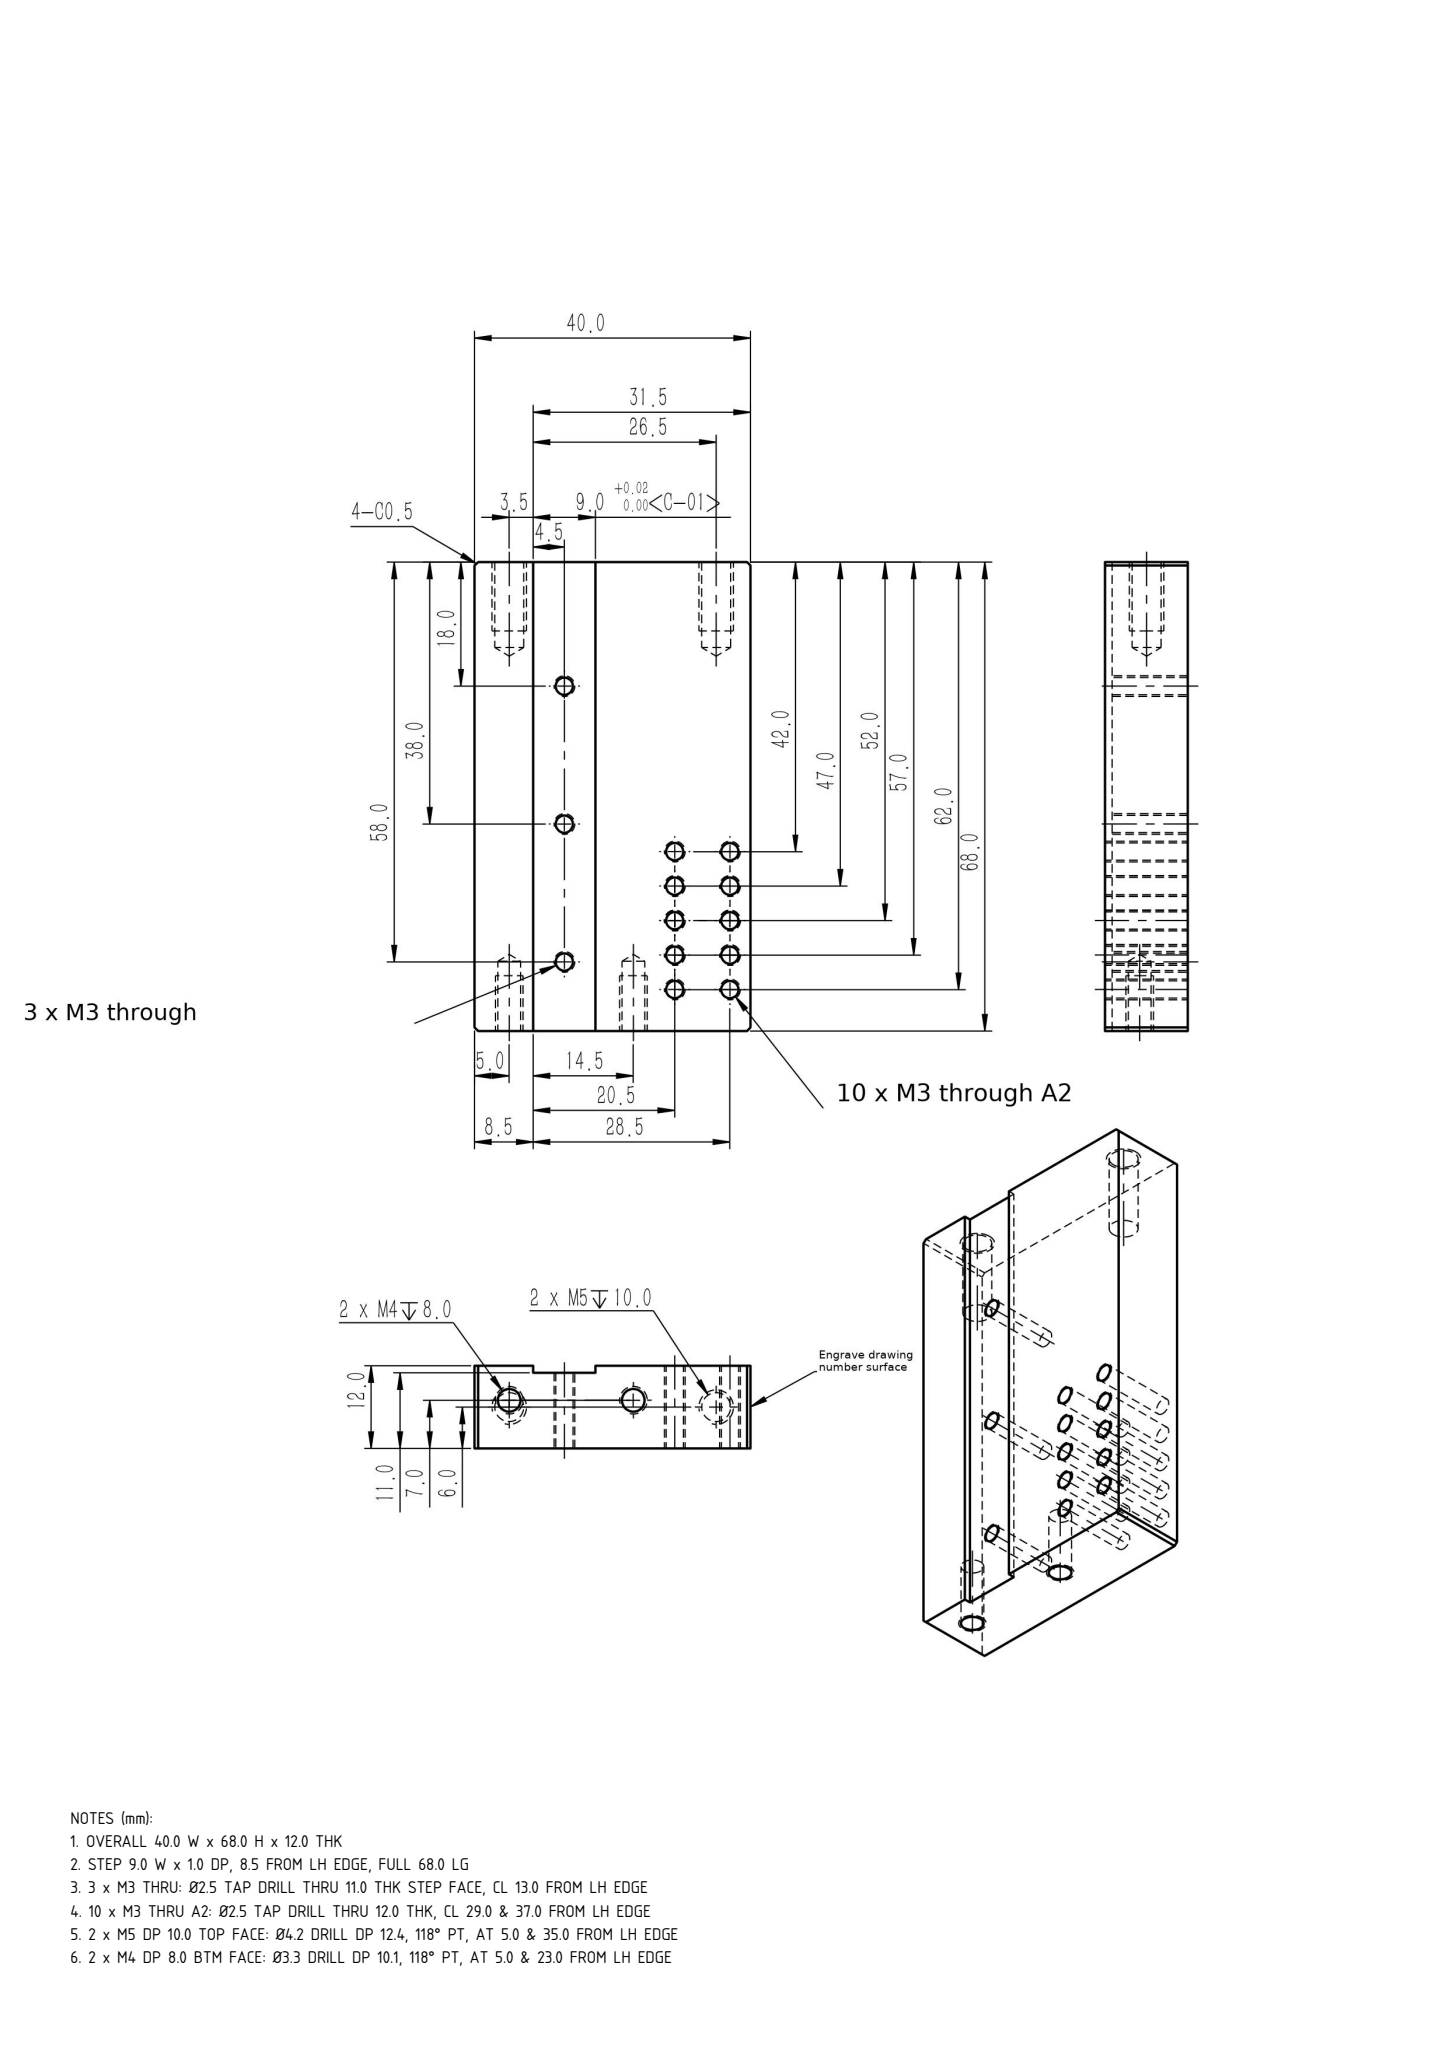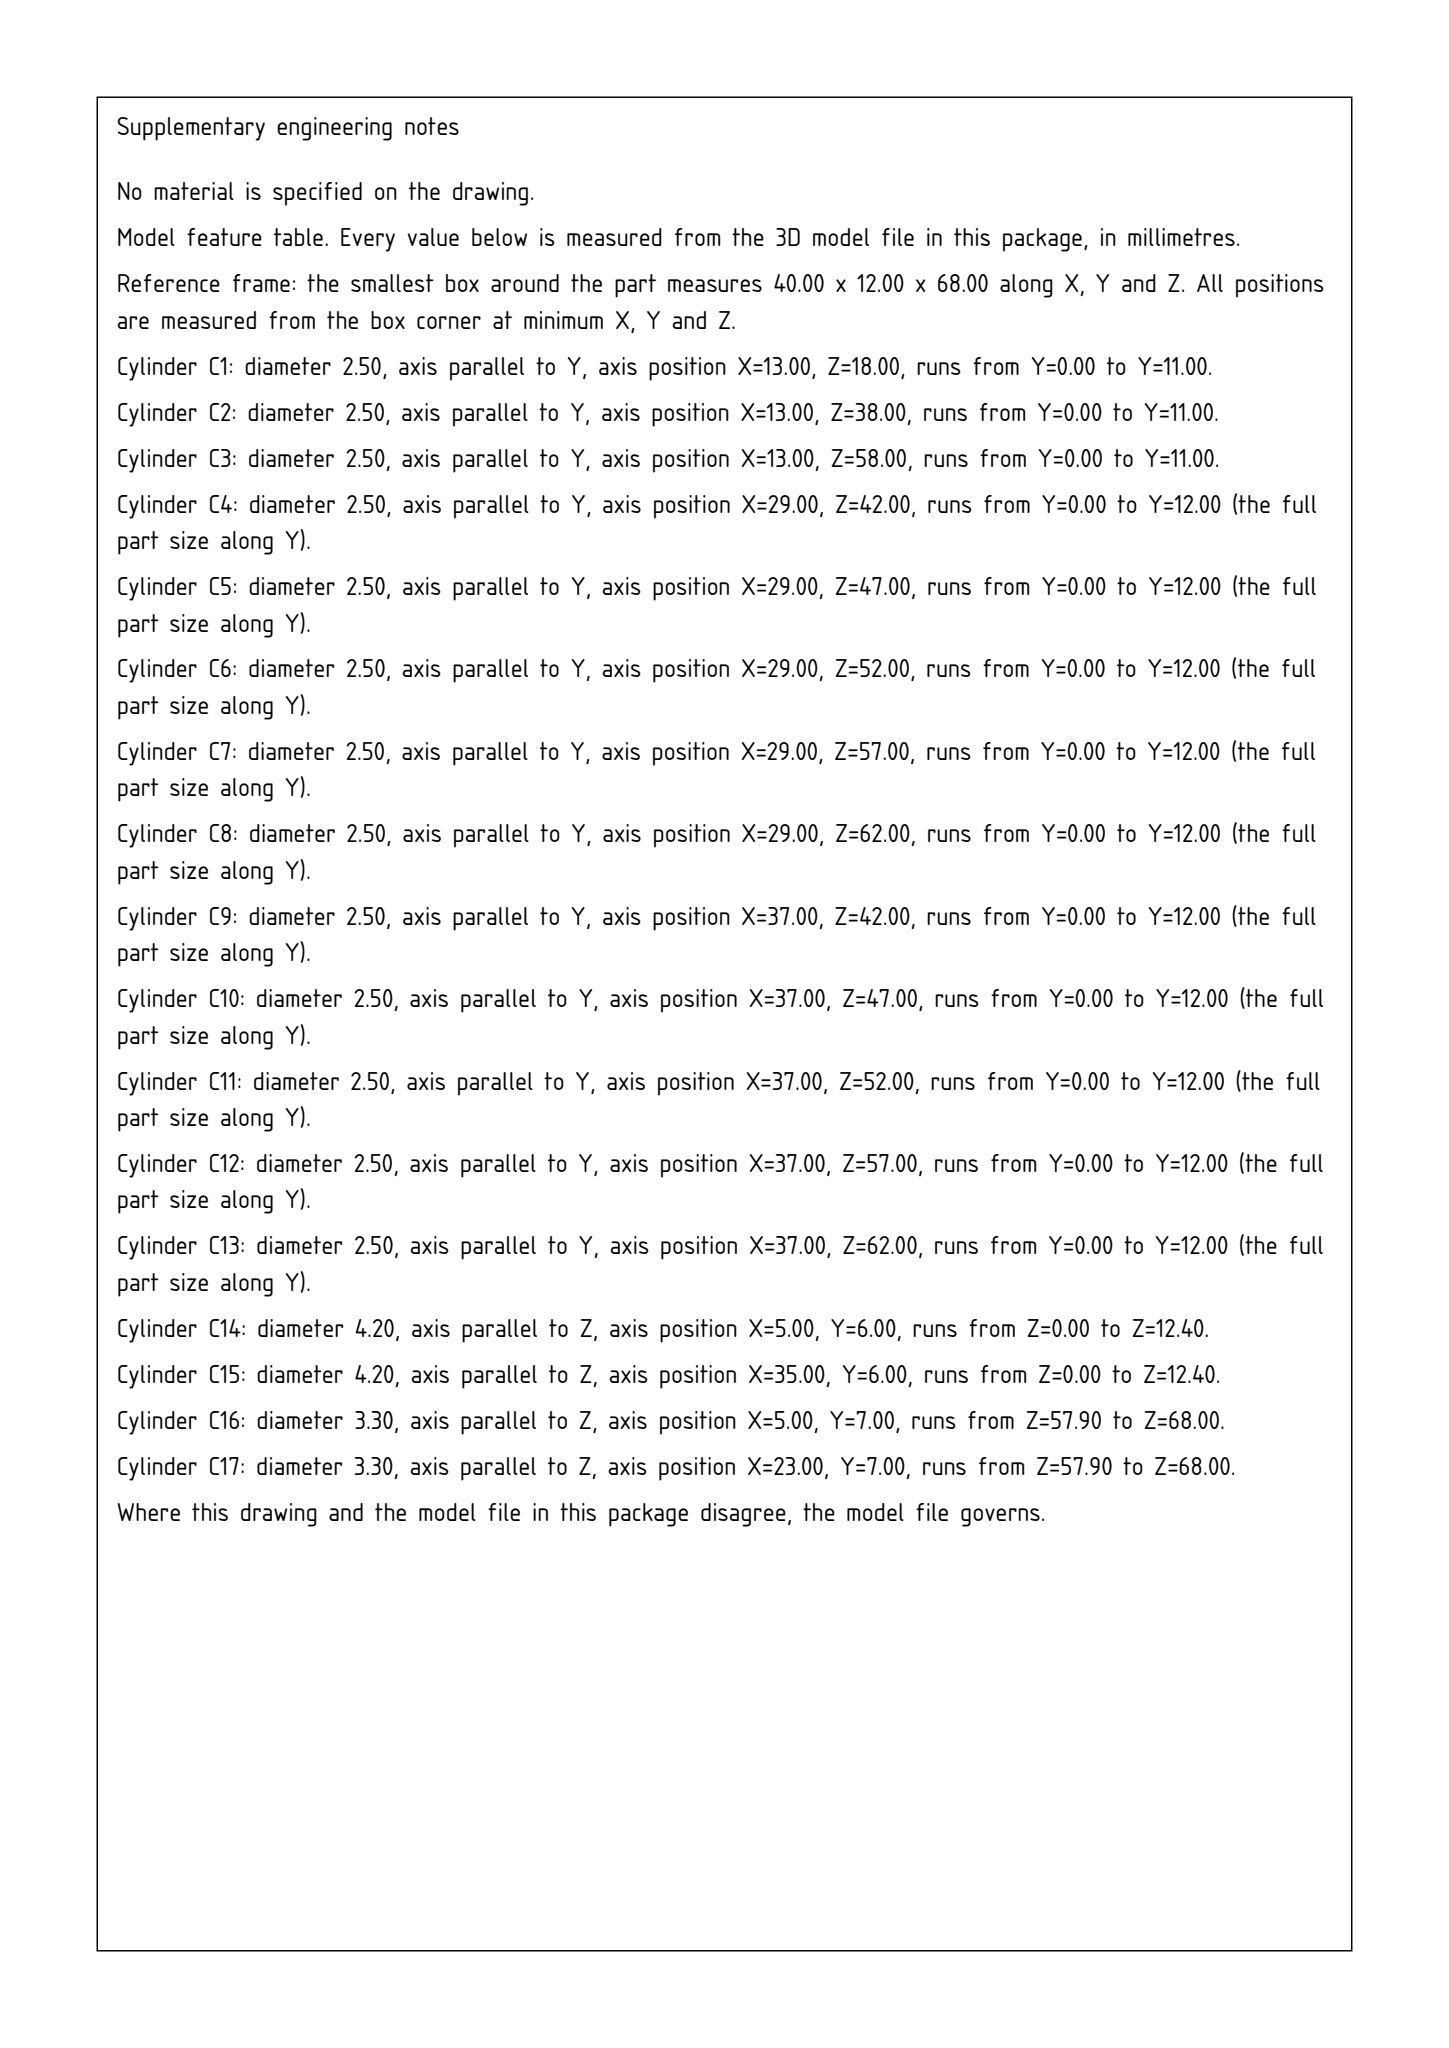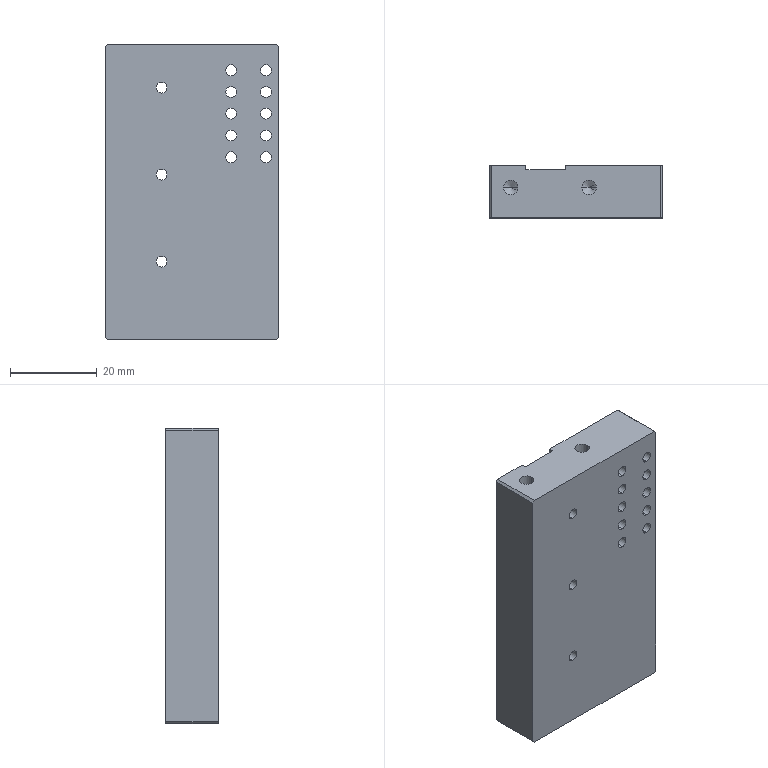Part | SolidWorks | mm | 1 solid | 56 faces | box 40 x 12 x 68 mm | volume 30737 mm3 | cylinder 34 | plane 14 | cone 8 | commonest cylinder face diameters 2.5 x26 3.3 x4 4.2 x4
Drawing notes:
OVERALL 40.0 W x 68.0 H x 12.0 THK | from the solid: bbox_xyz 40.0 x 12.0 x 68.0; planes x=0/40.0, y=0/12.0, z=0/68.0
STEP 9.0 W x 1.0 DP, 8.5 FROM LH EDGE, FULL 68.0 LG | from the solid: x-planes 8.5 & 17.5 (9.0 apart); y-planes 11.0 vs 12.0 = 1.0 DP; runs z=0 to 68.0
3 x M3 THRU: Ø2.5 TAP DRILL THRU 11.0 THK STEP FACE, CL 13.0 FROM LH EDGE | from the solid: Ø2.5 y-axis holes at x=13.0, z=18.0/38.0/58.0, length 11.0 (step floor y=11.0)
10 x M3 THRU A2: Ø2.5 TAP DRILL THRU 12.0 THK, CL 29.0 & 37.0 FROM LH EDGE | from the solid: Ø2.5 y-axis holes at x=29.0 & 37.0, z=42/47/52/57/62, length 12.0
2 x M5 DP 10.0 TOP FACE: Ø4.2 DRILL DP 12.4, 118° PT, AT 5.0 & 35.0 FROM LH EDGE | from the solid: Ø4.2 z-holes at (5.0,6.0) & (35.0,6.0), L=12.4 from z=68, 118° cone
2 x M4 DP 8.0 BTM FACE: Ø3.3 DRILL DP 10.1, 118° PT, AT 5.0 & 23.0 FROM LH EDGE | from the solid: Ø3.3 z-holes at (5.0,7.0) & (23.0,7.0), L=10.1 from z=0, 118° cone
build123d program:
from build123d import *

# Parameters (mm, degrees)
SKETCH1_W              = 40
SKETCH1_H              = 12
BOSS_EXTRUDE1_DEPTH    = 68
SKETCH2_W              = 9
SKETCH2_H              = 1
CUT_EXTRUDE1_DEPTH     = 80.8
M3_TAPPED_HOLE1_D      = 2.5
LPATTERN1_COUNT        = 3
LPATTERN1_PITCH        = 20
LPATTERN2_COUNT        = 2
LPATTERN2_PITCH        = 30
LPATTERN3_COUNT        = 2
LPATTERN3_PITCH        = 18
M3_TAPPED_HOLE2_D      = 2.5
LPATTERN4_COUNT        = 2
LPATTERN4_PITCH        = 8
LPATTERN5_COUNT        = 3
LPATTERN5_PITCH        = 5
LPATTERN5_COPY_1_D     = 2.5
LPATTERN5_COPY_2_D     = 2.5
LPATTERN5_COL_COUNT    = 3
LPATTERN5_COL_PITCH    = 5
LPATTERN5_COL_COPY_1_D = 2.5
LPATTERN5_COL_COPY_2_D = 2.5
CHAMFER1_SIZE          = 0.5


with BuildPart() as part:
    # Sketch1 → Boss-Extrude1 (new body)
    with BuildSketch(Plane.XY):
        with Locations((20, 6)):
            Rectangle(SKETCH1_W, SKETCH1_H)
    extrude(amount=BOSS_EXTRUDE1_DEPTH)

    # Sketch2 → Cut-Extrude1 (cut, through all)
    with BuildSketch(Plane.XY.offset(68)):
        with Locations((13, 11.5)):
            Rectangle(SKETCH2_W, SKETCH2_H)
    extrude(amount=-CUT_EXTRUDE1_DEPTH, mode=Mode.SUBTRACT)

    # M3 Tapped Hole1 (through all)
    with Locations(Plane(origin=(0, 11, 0), x_dir=(1, 0, 0), z_dir=(0, 1, 0))):
        with Locations((13, -58)):
            m3_tapped_hole1 = Hole(M3_TAPPED_HOLE1_D / 2)

    # LPattern1: M3 Tapped Hole1 ×3
    with Locations(*[(0, 0, -i * LPATTERN1_PITCH) for i in range(1, LPATTERN1_COUNT)]):
        add(m3_tapped_hole1, mode=Mode.SUBTRACT)

    # Sketch6 → M5 Tapped Hole2 (revolve, cut)
    with BuildSketch(Plane(origin=(5, 6, 0), x_dir=(0, 1, 0), z_dir=(1, 0, 0))):
        Polygon((0, 0), (0, 13.662), (2.1, 12.4), (2.1, 0), align=None)
    m5_tapped_hole2 = revolve(axis=Axis((5, 6, -6.35), (0, 0, 1)), mode=Mode.SUBTRACT)

    # LPattern2: M5 Tapped Hole2 ×2
    with Locations(*[(i * LPATTERN2_PITCH, 0, 0) for i in range(1, LPATTERN2_COUNT)]):
        add(m5_tapped_hole2, mode=Mode.SUBTRACT)

    # Sketch8 → M4 Tapped Hole1 (revolve, cut)
    with BuildSketch(Plane(origin=(5, 7, 68), x_dir=(0, -1, 0), z_dir=(1, 0, 0))):
        Polygon((0, 0), (0, 11.091), (1.65, 10.1), (1.65, 0), align=None)
    m4_tapped_hole1 = revolve(axis=Axis((5, 7, 74.35), (0, 0, -1)), mode=Mode.SUBTRACT)

    # LPattern3: M4 Tapped Hole1 ×2
    with Locations(*[(i * LPATTERN3_PITCH, 0, 0) for i in range(1, LPATTERN3_COUNT)]):
        add(m4_tapped_hole1, mode=Mode.SUBTRACT)

    # M3 Tapped Hole2 (through all)
    with Locations(Plane(origin=(0, 12, 0), x_dir=(1, 0, 0), z_dir=(0, 1, 0))):
        with Locations((37, -52)):
            m3_tapped_hole2 = Hole(M3_TAPPED_HOLE2_D / 2)

    # LPattern4: M3 Tapped Hole2 ×2
    with Locations(*[(-i * LPATTERN4_PITCH, 0, 0) for i in range(1, LPATTERN4_COUNT)]):
        add(m3_tapped_hole2, mode=Mode.SUBTRACT)

    # LPattern5: M3 Tapped Hole2 ×3
    with Locations(*[(0, 0, i * LPATTERN5_PITCH) for i in range(1, LPATTERN5_COUNT)]):
        add(m3_tapped_hole2, mode=Mode.SUBTRACT)

    # LPattern5 copy 1 (through all)
    with Locations(Plane(origin=(-8, 12, 5), x_dir=(1, 0, 0), z_dir=(0, 1, 0))):
        with Locations((37, -52)):
            Hole(LPATTERN5_COPY_1_D / 2)

    # LPattern5 copy 2 (through all)
    with Locations(Plane(origin=(-8, 12, 10), x_dir=(1, 0, 0), z_dir=(0, 1, 0))):
        with Locations((37, -52)):
            Hole(LPATTERN5_COPY_2_D / 2)

    # LPattern5 col: M3 Tapped Hole2 ×3
    with Locations(*[(0, 0, -i * LPATTERN5_COL_PITCH) for i in range(1, LPATTERN5_COL_COUNT)]):
        add(m3_tapped_hole2, mode=Mode.SUBTRACT)

    # LPattern5 col copy 1 (through all)
    with Locations(Plane(origin=(-8, 12, -5), x_dir=(1, 0, 0), z_dir=(0, 1, 0))):
        with Locations((37, -52)):
            Hole(LPATTERN5_COL_COPY_1_D / 2)

    # LPattern5 col copy 2 (through all)
    with Locations(Plane(origin=(-8, 12, -10), x_dir=(1, 0, 0), z_dir=(0, 1, 0))):
        with Locations((37, -52)):
            Hole(LPATTERN5_COL_COPY_2_D / 2)

    # Chamfer1
    chamfer1_edges = [part.edges().sort_by_distance(p)[0] for p in [
        (40, 6, 68),
        (0, 6, 68),
        (40, 6, 0),
        (0, 6, 0),
    ]]
    chamfer(chamfer1_edges, length=CHAMFER1_SIZE)


solid = part.part